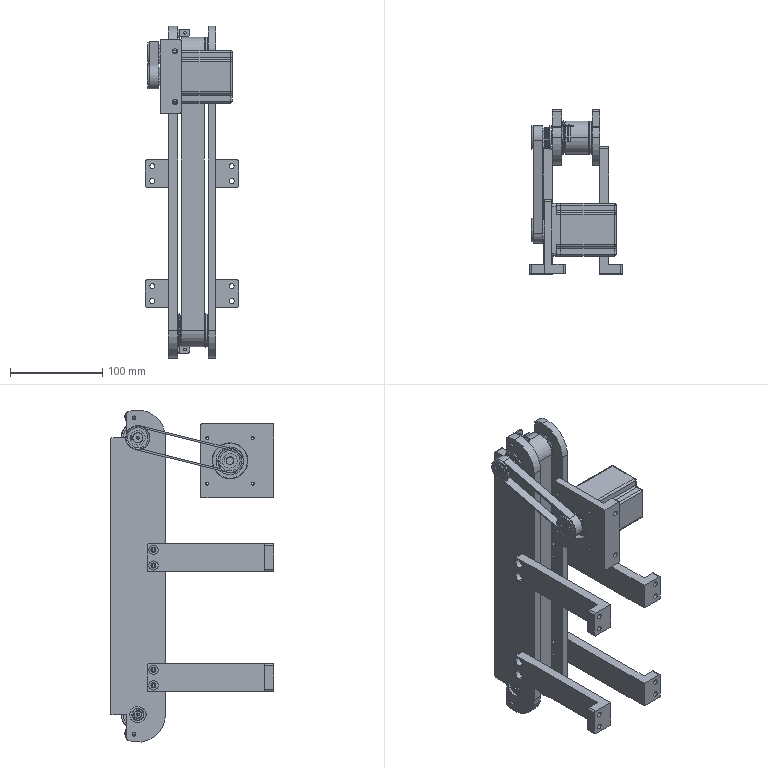Assembly | SolidWorks | mm | 24 component files | 25 solids | 1722 faces | box 101 x 177.5 x 360 mm | volume 881601 mm3 | cylinder 1064 | plane 260 | cone 250 | spline 128 | torus 12 | sphere 8 | commonest cylinder face diameters 1.1 x168 0.5 x164 6.55 x156 4 x84 10 x48 27.33 x46 30.87 x40 5.5 x36
Bill of materials:
57Stepper | 1 |  | Square-section prismatic body with a thin square front flange with rounded corners, a hole in each corner, and one cylindrical shaft sticking out of the flange face. Corner notches with rounded edges run the full length of the body.
BAF608ZZ | 4 |  | Short annular cylinder (ring) with a central through-bore. Each face has concentric stepped rings, like a radial bearing with shields.
DCRSW-310-ReflectionFiber | 2 |  | Solid cylindrical rod with a short, smaller-diameter stepped section at one end.
EBJ22-S5M150-14-A-H-d10 | 1 |  | Toothed cylindrical pulley with a raised flange at each end and a central bore with a single keyway.
EBJ22-S5M150-14-A-H-d8 | 1 |  | Toothed flanged pulley that looks almost the same as the previous pulley, with a central bore and a single keyway. The keyway is set at a different angle and the bore looks smaller.
EBJ41-S5M250-20-A-N-d10 | 2 |  | Wider toothed flanged pulley with more teeth, a central bore with a keyway, and one radial hole through the toothed hub.
RearConveyorLine,Width17mm | 1 |  | Closed loop shaped like a thin-walled obround (stadium) band, with uniform width and smooth, untoothed surfaces.
RearConveyorLine,Width27mm | 1 |  | Closed, thin-walled obround (stadium) band loop that is long and narrow, with a wide band width compared with the loop's span.
ZHDJ-A0017 | 2 |  | L-shaped bent plate bracket with a rounded inside bend. Each leg has one round through-hole. One leg has a curved, tapered outer edge.
ZHDJ-G001 | 1 |  | Long thin flat plate with rounded ends. Each end has a through-hole and a rectangular step notch. Pairs of very small holes or marks sit along the plate.
ZHDJ-G002 | 4 |  | Long bar with an L-shaped cross-section: a tall web with a short perpendicular foot along one edge. Each end has a pair of through-holes.
ZHDJ-G003 | 1 |  | L-profile plate with a large central circular opening, four small holes in a square pattern around it, and a short perpendicular flange along one edge that has two holes.
ZHDJ-G004 | 1 |  | Solid stepped cylindrical shaft with five coaxial sections of different diameters: a large section at one end, a short shoulder, a reduced neck, a long middle section, and a smaller end journal. Two elongated slots with rounded ends, likely keyways, sit on the large end section and the long middle section. One end face has a small central recess with a conical bottom.
ZHDJ-G005 | 1 |  | Solid stepped cylindrical shaft with three coaxial sections: a long, larger-diameter middle section between two smaller-diameter end journals of similar length. One shallow slot with rounded ends, likely a keyway, runs along most of the middle section. The visible end face has a small central recess with a conical bottom.
ZHDJ-G006 | 1 |  | Thin, elongated, flat plate. One long edge is straight with rounded corners at both ends, and the other long edge has a stepped profile: a narrower tab at each end and a wider straight-edged central region. Each end tab has a larger round through-hole, which may be countersunk or chamfered. There are also several small holes: one near each end tip and two pairs spaced along the length near the straight edge.
Mates:
1. distance | ZHDJ-G006-1 face at (5, 0, 150) dir (1, 0, 0) | ZHDJ-G001-2 face at (38, 0, 150) dir (-1, 0, 0)
2. coincident | ZHDJ-G006-1 face at (5, 30, 150) dir (0, 1, 0) | ZHDJ-G001-2 face at (46, 30, 150) dir (0, 1, 0)
3. concentric | ZHDJ-G006-1 face at (5, 0, 150) dir (-1, 0, 0) r 30 | ZHDJ-G001-2 face at (46, 0, 150) dir (-1, 0, 0) r 30
4. coincident | ZHDJ-G001-2 face at (46, 0, 150) dir (1, 0, 0) | ZHDJ-G002-1 face at (46, -137.498, -95) dir (-1, 0, 0)
5. concentric | ZHDJ-G006-1 face at (-5, 0, 150) dir (1, 0, 0) r 9 | EBJ22-S5M150-14-A-H-d10-3 face at (-28, 0, 150) dir (1, 0, 0) r 5.5
6. concentric | ZHDJ-G001-2 face at (36, 0, 150) dir (1, 0, 0) r 9 | ZHDJ-G004-1 face at (37, 0, 150) dir (-1, 0, 0) r 5
7. concentric | ZHDJ-G006-1 face at (-5, 0, -150) dir (1, 0, 0) r 9 | ZHDJ-G005-1 face at (36, 0, -150) dir (-1, 0, 0) r 5
8. width | ZHDJ-G001-2 face at (46, 0, 150) dir (1, 0, 0) | ZHDJ-G006-1 face at (-5, 0, 150) dir (-1, 0, 0) | ZHDJ-G005-1 face at (36, 0, -150) dir (1, 0, 0) | ZHDJ-G005-1 face at (5, 0, -150) dir (-1, 0, 0)
9. coincident | ZHDJ-G001-2 face at (38, 0, 150) dir (-1, 0, 0) | BAF608ZZ-1 face at (38, 6, 150) dir (-1, 0, 0)
10. concentric | ZHDJ-G004-1 face at (37, 0, 150) dir (-1, 0, 0) r 5 | BAF608ZZ-2 face at (4.7, 0, 150) dir (-1, 0, 0) r 4
11. coincident | ZHDJ-G006-1 face at (5, 0, 150) dir (1, 0, 0) | BAF608ZZ-2 face at (5, 9.75, 150) dir (1, 0, 0)
12. concentric | ZHDJ-G005-1 face at (36, 0, -150) dir (-1, 0, 0) r 5 | BAF608ZZ-3 face at (44.7, 0, -150) dir (-1, 0, 0) r 4
13. coincident | ZHDJ-G001-2 face at (38, 0, 150) dir (-1, 0, 0) | BAF608ZZ-3 face at (38, -10.347, -147.274) dir (-1, 0, 0)
14. concentric | ZHDJ-G005-1 face at (36, 0, -150) dir (-1, 0, 0) r 5 | BAF608ZZ-4 face at (4.7, 0, -150) dir (-1, 0, 0) r 4
15. coincident | ZHDJ-G006-1 face at (5, 0, 150) dir (1, 0, 0) | BAF608ZZ-4 face at (5, 9.567, -151.88) dir (1, 0, 0)
16. concentric | ZHDJ-G004-1 face at (-28, 0, 150) dir (1, 0, 0) r 5.5 | RearConveyorLine,Width17mm-1 face at (-15.5, 0, 150) dir (-1, 0, 0) r 13.14
17. concentric | ZHDJ-G005-1 face at (36, 0, -150) dir (-1, 0, 0) r 5 | RearConveyorLine,Width27mm-1 face at (34, 0, -150) dir (-1, 0, 0) r 17.92
18. concentric | ZHDJ-G004-1 face at (37, 0, 150) dir (-1, 0, 0) r 5 | RearConveyorLine,Width27mm-1 face at (34, 0, 150) dir (-1, 0, 0) r 17.92
19. width | ZHDJ-G006-1 face at (5, 0, 150) dir (1, 0, 0) | ZHDJ-G001-2 face at (38, 0, 150) dir (-1, 0, 0) | RearConveyorLine,Width27mm-1 face at (34, 0, -150) dir (1, 0, 0) | RearConveyorLine,Width27mm-1 face at (9, 0, -150) dir (-1, 0, 0)
20. concentric | BAF608ZZ-3 face at (44.7, 0, -150) dir (-1, 0, 0) r 11 | ZHDJ-G001-2 face at (36, 0, -150) dir (1, 0, 0) r 9
21. concentric | EBJ22-S5M150-14-A-H-d10-3 face at (-28, 0, 150) dir (1, 0, 0) r 5.5 | ZHDJ-G004-1 face at (37, 0, 150) dir (-1, 0, 0) r 5
22. concentric | ZHDJ-G004-1 face at (37, 0, 150) dir (-1, 0, 0) r 5 | BAF608ZZ-1 face at (44.7, 0, 150) dir (-1, 0, 0) r 4
23. concentric | ZHDJ-G006-1 face at (-5, -17.002, -118.5) dir (-1, 0, 0) r 2.1 | ZHDJ-G002-2 face at (-15, -17.002, -118.5) dir (-1, 0, 0) r 5
24. concentric | ZHDJ-G006-1 face at (-5, -17.002, -101.5) dir (-1, 0, 0) r 2.1 | ZHDJ-G002-2 face at (-15, -17.002, -101.5) dir (-1, 0, 0) r 2.75
25. concentric | ZHDJ-G001-2 face at (46, -17, -118.5) dir (1, 0, 0) r 2.1 | ZHDJ-G002-1 face at (56, -17, -118.5) dir (1, 0, 0) r 5
26. concentric | ZHDJ-A0017-1 face at (13, 21.5, 172.5) dir (0, -1, 0) r 1.5 | DCRSW-310-ReflectionFiber-1 face at (13, -4, 172.5) dir (0, 1, 0) r 1.45
27. coincident | ZHDJ-A0017-1 face at (5, 13, 168.5) dir (0, 1, 0) | DCRSW-310-ReflectionFiber-1 face at (13, 13, 172.5) dir (0, 1, 0)
28. concentric | ZHDJ-A0017-4 face at (13, 21.5, -170.5) dir (0, -1, 0) r 1.5 | DCRSW-310-ReflectionFiber-2 face at (13, -4, -170.5) dir (0, 1, 0) r 1.45
29. coincident | ZHDJ-A0017-4 face at (5, 13, -174.5) dir (0, 1, 0) | DCRSW-310-ReflectionFiber-2 face at (13, 13, -170.5) dir (0, 1, 0)
30. concentric | 57Stepper-1 face at (-28, -99.859, 124.987) dir (1, 0, 0) r 4 | EBJ22-S5M150-14-A-H-d8-1 face at (-28, -99.859, 124.987) dir (1, 0, 0) r 4
31. coincident | EBJ22-S5M150-14-A-H-d10-3 face at (-28, 8, 150.018) dir (-1, 0, 0) | EBJ22-S5M150-14-A-H-d8-1 face at (-28, -92.166, 127.182) dir (-1, 0, 0)
32. coincident | 57Stepper-1 face at (-28, -99.859, 124.987) dir (-1, 0, 0) | EBJ22-S5M150-14-A-H-d8-1 face at (-28, -92.166, 127.182) dir (-1, 0, 0)
33. distance | EBJ22-S5M150-14-A-H-d10-3 face at (-6, 0, 150) dir (1, 0, 0) | ZHDJ-G006-1 face at (-5, 0, 150) dir (-1, 0, 0)
34. coincident | EBJ22-S5M150-14-A-H-d10-3 face at (-28, 8, 150.018) dir (-1, 0, 0) | EBJ22-S5M150-14-A-H-d8-1 face at (-28, -92.166, 127.182) dir (-1, 0, 0)
35. concentric | ZHDJ-G003-1 face at (6, -99.859, 124.987) dir (-1, 0, 0) r 19.5 | 57Stepper-1 face at (-28, -99.859, 124.987) dir (1, 0, 0) r 4
36. coincident | ZHDJ-G003-1 face at (-6, -107.5, 124.987) dir (1, 0, 0) | 57Stepper-1 face at (-6, -99.859, 124.987) dir (-1, 0, 0)
37. coincident | RearConveyorLine,Width17mm-1 face at (-25.5, 0, 150) dir (-1, 0, 0) | EBJ22-S5M150-14-A-H-d8-1 face at (-25.5, -89.127, 128.049) dir (1, 0, 0)
38. coincident | ZHDJ-G006-1 face at (5, 0, 150) dir (1, 0, 0) | ZHDJ-A0017-1 face at (5, 11.5, 172.5) dir (-1, 0, 0)
39. parallel | ZHDJ-G006-1 face at (-15, 30, 150) dir (0, 0, 1) | ZHDJ-A0017-1 face at (5, 11.5, 176.5) dir (0, 0, 1)
40. concentric | ZHDJ-G006-1 face at (-5, 4, 171.5) dir (1, 0, 0) r 2 | ZHDJ-A0017-1 face at (15, 4, 171.5) dir (-1, 0, 0) r 2.5
41. concentric | ZHDJ-G006-1 face at (-5, 4, -171.5) dir (1, 0, 0) r 2 | ZHDJ-A0017-4 face at (15, 4, -171.5) dir (-1, 0, 0) r 2.5
42. parallel | ZHDJ-G006-1 face at (-15, 30, -150) dir (0, 0, -1) | ZHDJ-A0017-4 face at (5, -2, -174.5) dir (0, 0, -1)
43. coincident | ZHDJ-G006-1 face at (5, 0, 150) dir (1, 0, 0) | ZHDJ-A0017-4 face at (5, 11.5, -170.5) dir (-1, 0, 0)
44. parallel | ZHDJ-G003-1 face at (-6, -67.5, 164.987) dir (0, 0, 1) | 57Stepper-1 face at (64, -83.359, 153.487) dir (0, 0, 1)
45. coincident | ZHDJ-G003-1 face at (-6, -147.5, 164.987) dir (0, -1, 0) | ZHDJ-G002-6 face at (-15, -147.5, 5) dir (0, -1, 0)
46. coincident | EBJ22-S5M150-14-A-H-d10-3 face at (-28, 8, 150.018) dir (-1, 0, 0) | ZHDJ-G004-1 face at (-28, 0, 150) dir (-1, 0, 0)